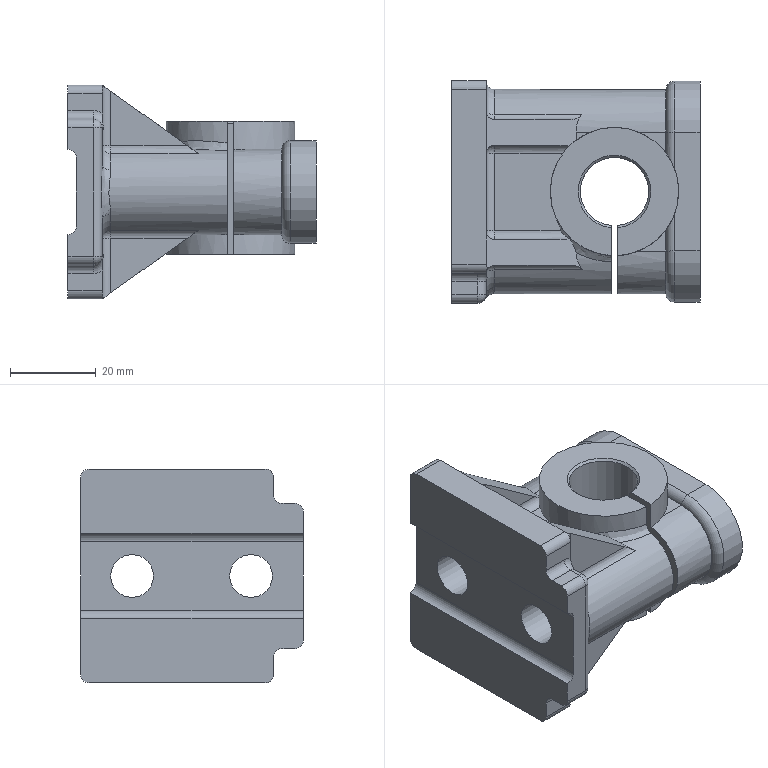Component | NX | ROCKER_ARM_SHAFT_SEAT | 1 solid | 107 faces | volume 58270 mm3 | plane 44 | cylinder 44 | torus 8 | sphere 8 | spline 2 | cone 1 | commonest cylinder face diameters 4 x32 20 x3 10 x3 30 x2 24 x2 22 x1 16 x1